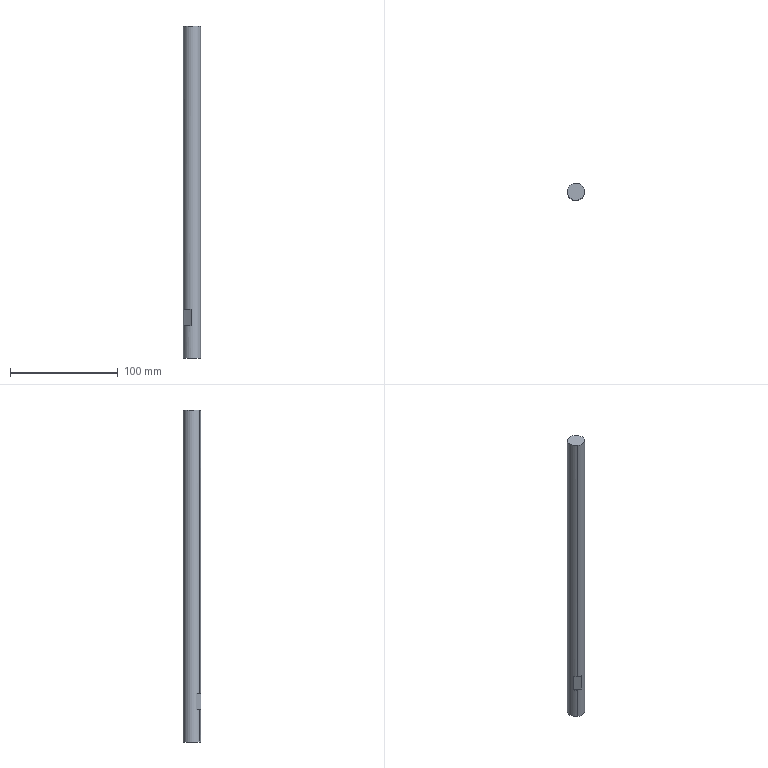Component | SolidWorks | SupportRod-1 | 1 solid | 16 faces | box 16 x 16 x 308 mm | volume 60860 mm3 | plane 8 | cone 4 | cylinder 4 | commonest cylinder face diameters 6.8 x2 16 x2
build123d program:
from build123d import *

# Parameters (mm, degrees)
SKETCH1_W                                            = 8
SKETCH1_H                                            = 308
CUT_EXTRUDE1_DEPTH                                   = 15
CUT_EXTRUDE2_START                                   = -15
CUT_EXTRUDE2_DEPTH                                   = 15
M6_FLAT_HEAD_MACHINE_SCREW_COUNTERSUNK_H_D           = 6.8
M6_FLAT_HEAD_MACHINE_SCREW_COUNTERSUNK_H_DEPTH       = 24.25
M6_FLAT_HEAD_MACHINE_SCREW_COUNTERSUNK_H_CSINK_D     = 8.05
M6_FLAT_HEAD_MACHINE_SCREW_COUNTERSUNK_H_CSINK_ANGLE = 90
M6_FLAT_HEAD_MACHINE_SCREW_COUNTERSUNK_H_TIP         = 2.043


with BuildPart() as part:
    # Sketch1 → Revolve1 (revolve)
    with BuildSketch(Plane.XZ, mode=Mode.PRIVATE) as revolve1_sk:
        with Locations((4, 0)):
            Rectangle(SKETCH1_W, SKETCH1_H)
    revolve(revolve1_sk.sketch.rotate(Axis((0, 0, 154), (0, 0, -1)), 180), axis=Axis((0, 0, 154), (0, 0, -1)))

    # Sketch2 → Cut-Extrude1 (cut)
    with BuildSketch(Plane.XY.offset(124)):
        with BuildLine():
            Line((7, 3.873), (7, -3.873))
            ThreePointArc((7, -3.873), (8, 0), (7, 3.873))
        make_face()
    extrude(amount=-CUT_EXTRUDE1_DEPTH, mode=Mode.SUBTRACT)

    # Sketch3 → Cut-Extrude2 (cut)
    with BuildSketch(Plane(origin=(0, 0, 109), x_dir=(-1, 0, 0), z_dir=(0, 0, -1)).offset(CUT_EXTRUDE2_START)):
        with BuildLine():
            Line((7, 3.873), (7, -3.873))
            ThreePointArc((7, -3.873), (8, 0), (7, 3.873))
        make_face()
    extrude(amount=CUT_EXTRUDE2_DEPTH, mode=Mode.SUBTRACT)

    # M6 Flat Head Machine Screw Countersunk H
    with Locations(Plane.XY.offset(154)):
        with Locations((0, 0)):
            CounterSinkHole(M6_FLAT_HEAD_MACHINE_SCREW_COUNTERSUNK_H_D / 2, M6_FLAT_HEAD_MACHINE_SCREW_COUNTERSUNK_H_CSINK_D / 2, depth=M6_FLAT_HEAD_MACHINE_SCREW_COUNTERSUNK_H_DEPTH, counter_sink_angle=M6_FLAT_HEAD_MACHINE_SCREW_COUNTERSUNK_H_CSINK_ANGLE)
            with Locations((0, 0, -(M6_FLAT_HEAD_MACHINE_SCREW_COUNTERSUNK_H_DEPTH + M6_FLAT_HEAD_MACHINE_SCREW_COUNTERSUNK_H_TIP / 2))):  # 118° drill point
                Cone(0, M6_FLAT_HEAD_MACHINE_SCREW_COUNTERSUNK_H_D / 2, M6_FLAT_HEAD_MACHINE_SCREW_COUNTERSUNK_H_TIP, mode=Mode.SUBTRACT)


solid = part.part

# Placed as in the assembly
solid = solid.moved(Location((-100, -212, -108.5), (180, 0, 125.085)))
STEP:
#1=COLOUR_RGB('',0.7922,0.8196,0.9333);
#2=FILL_AREA_STYLE_COLOUR('',#1);
#3=FILL_AREA_STYLE('',(#2));
#4=SURFACE_STYLE_FILL_AREA(#3);
#5=SURFACE_SIDE_STYLE('',(#4));
#6=SURFACE_STYLE_USAGE(.BOTH.,#5);
#7=PRESENTATION_STYLE_ASSIGNMENT((#6));
#8=CARTESIAN_POINT('',(-3.86,-8.237,-10.31));
#9=VERTEX_POINT('',#8);
#10=CARTESIAN_POINT('',(-4.014,-8.456,-10.31));
#11=VERTEX_POINT('',#10);
#12=CARTESIAN_POINT('',(-3.937,-8.346,-10.31));
#13=DIRECTION('',(0.,0.,-1.));
#14=DIRECTION('',(-0.5748,-0.8183,0.));
#15=AXIS2_PLACEMENT_3D('',#12,#13,#14);
#16=CIRCLE('',#15,0.1339);
#17=EDGE_CURVE('',#9,#11,#16,.T.);
#18=ORIENTED_EDGE('',*,*,#17,.F.);
#19=CARTESIAN_POINT('',(-3.846,-8.217,-10.335));
#20=VERTEX_POINT('',#19);
#21=CARTESIAN_POINT('',(-3.846,-8.217,-10.335));
#22=DIRECTION('',(0.4064,0.5786,-0.7071));
#23=VECTOR('',#22,39.37);
#24=LINE('',#21,#23);
#25=EDGE_CURVE('',#9,#20,#24,.T.);
#26=ORIENTED_EDGE('',*,*,#25,.T.);
#27=CARTESIAN_POINT('',(-4.028,-8.476,-10.335));
#28=VERTEX_POINT('',#27);
#29=CARTESIAN_POINT('',(-3.937,-8.346,-10.335));
#30=DIRECTION('',(0.,0.,-1.));
#31=DIRECTION('',(-0.5748,-0.8183,0.));
#32=AXIS2_PLACEMENT_3D('',#29,#30,#31);
#33=CIRCLE('',#32,0.1585);
#34=EDGE_CURVE('',#20,#28,#33,.T.);
#35=ORIENTED_EDGE('',*,*,#34,.T.);
#36=CARTESIAN_POINT('',(-4.028,-8.476,-10.335));
#37=DIRECTION('',(-0.4064,-0.5786,-0.7071));
#38=VECTOR('',#37,39.37);
#39=LINE('',#36,#38);
#40=EDGE_CURVE('',#11,#28,#39,.T.);
#41=ORIENTED_EDGE('',*,*,#40,.F.);
#42=EDGE_LOOP('',(#18,#26,#35,#41));
#43=FACE_OUTER_BOUND('',#42,.T.);
#44=CARTESIAN_POINT('',(-3.937,-8.346,-10.335));
#45=DIRECTION('',(0.,0.,-1.));
#46=DIRECTION('',(-0.5748,-0.8183,0.));
#47=AXIS2_PLACEMENT_3D('',#44,#45,#46);
#48=CONICAL_SURFACE('',#47,0.1585,0.7854);
#49=ADVANCED_FACE('',(#43),#48,.F.);
#50=CARTESIAN_POINT('',(-3.86,-8.237,-9.38));
#51=VERTEX_POINT('',#50);
#52=CARTESIAN_POINT('',(-4.014,-8.456,-9.38));
#53=VERTEX_POINT('',#52);
#54=CARTESIAN_POINT('',(-3.937,-8.346,-9.38));
#55=DIRECTION('',(0.,0.,-1.));
#56=DIRECTION('',(-0.5748,-0.8183,0.));
#57=AXIS2_PLACEMENT_3D('',#54,#55,#56);
#58=CIRCLE('',#57,0.1339);
#59=EDGE_CURVE('',#51,#53,#58,.T.);
#60=ORIENTED_EDGE('',*,*,#59,.F.);
#61=CARTESIAN_POINT('',(-3.86,-8.237,-10.335));
#62=DIRECTION('',(0.,0.,-1.));
#63=VECTOR('',#62,39.37);
#64=LINE('',#61,#63);
#65=EDGE_CURVE('',#51,#9,#64,.T.);
#66=ORIENTED_EDGE('',*,*,#65,.T.);
#67=ORIENTED_EDGE('',*,*,#17,.T.);
#68=CARTESIAN_POINT('',(-4.014,-8.456,-10.335));
#69=DIRECTION('',(0.,0.,-1.));
#70=VECTOR('',#69,39.37);
#71=LINE('',#68,#70);
#72=EDGE_CURVE('',#53,#11,#71,.T.);
#73=ORIENTED_EDGE('',*,*,#72,.F.);
#74=EDGE_LOOP('',(#60,#66,#67,#73));
#75=FACE_OUTER_BOUND('',#74,.T.);
#76=CARTESIAN_POINT('',(-3.937,-8.346,-10.335));
#77=DIRECTION('',(0.,0.,-1.));
#78=DIRECTION('',(-0.5748,-0.8183,0.));
#79=AXIS2_PLACEMENT_3D('',#76,#77,#78);
#80=CYLINDRICAL_SURFACE('',#79,0.1339);
#81=ADVANCED_FACE('',(#75),#80,.F.);
#82=CARTESIAN_POINT('',(-3.937,-8.346,-9.299));
#83=VERTEX_POINT('',#82);
#84=CARTESIAN_POINT('',(-4.014,-8.456,-9.38));
#85=DIRECTION('',(-0.4927,-0.7014,-0.515));
#86=VECTOR('',#85,39.37);
#87=LINE('',#84,#86);
#88=EDGE_CURVE('',#83,#53,#87,.T.);
#89=ORIENTED_EDGE('',*,*,#88,.F.);
#90=CARTESIAN_POINT('',(-3.86,-8.237,-9.38));
#91=DIRECTION('',(0.4927,0.7014,-0.515));
#92=VECTOR('',#91,39.37);
#93=LINE('',#90,#92);
#94=EDGE_CURVE('',#83,#51,#93,.T.);
#95=ORIENTED_EDGE('',*,*,#94,.T.);
#96=ORIENTED_EDGE('',*,*,#59,.T.);
#97=EDGE_LOOP('',(#89,#95,#96));
#98=FACE_OUTER_BOUND('',#97,.T.);
#99=CARTESIAN_POINT('',(-3.937,-8.346,-9.38));
#100=DIRECTION('',(0.,0.,-1.));
#101=DIRECTION('',(-0.5748,-0.8183,0.));
#102=AXIS2_PLACEMENT_3D('',#99,#100,#101);
#103=CONICAL_SURFACE('',#102,0.1339,1.03);
#104=ADVANCED_FACE('',(#98),#103,.F.);
#105=CARTESIAN_POINT('',(-3.756,-8.089,-10.335));
#106=VERTEX_POINT('',#105);
#107=CARTESIAN_POINT('',(-4.118,-8.604,-10.335));
#108=VERTEX_POINT('',#107);
#109=CARTESIAN_POINT('',(-3.937,-8.346,-10.335));
#110=DIRECTION('',(-0.,0.,1.));
#111=DIRECTION('',(0.5748,0.8183,0.));
#112=AXIS2_PLACEMENT_3D('',#109,#110,#111);
#113=CIRCLE('',#112,0.315);
#114=EDGE_CURVE('',#106,#108,#113,.T.);
#115=ORIENTED_EDGE('',*,*,#114,.T.);
#116=CARTESIAN_POINT('',(-4.118,-8.604,-9.154));
#117=VERTEX_POINT('',#116);
#118=CARTESIAN_POINT('',(-4.118,-8.604,-10.335));
#119=DIRECTION('',(-0.,0.,1.));
#120=VECTOR('',#119,39.37);
#121=LINE('',#118,#120);
#122=EDGE_CURVE('',#108,#117,#121,.T.);
#123=ORIENTED_EDGE('',*,*,#122,.T.);
#124=CARTESIAN_POINT('',(-4.22,-8.484,-9.154));
#125=VERTEX_POINT('',#124);
#126=CARTESIAN_POINT('',(-3.937,-8.346,-9.154));
#127=DIRECTION('',(0.,0.,-1.));
#128=DIRECTION('',(-0.5748,-0.8183,0.));
#129=AXIS2_PLACEMENT_3D('',#126,#127,#128);
#130=CIRCLE('',#129,0.315);
#131=EDGE_CURVE('',#117,#125,#130,.T.);
#132=ORIENTED_EDGE('',*,*,#131,.T.);
#133=CARTESIAN_POINT('',(-4.22,-8.484,-8.563));
#134=VERTEX_POINT('',#133);
#135=CARTESIAN_POINT('',(-4.22,-8.484,-8.563));
#136=DIRECTION('',(0.,0.,-1.));
#137=VECTOR('',#136,39.37);
#138=LINE('',#135,#137);
#139=EDGE_CURVE('',#134,#125,#138,.T.);
#140=ORIENTED_EDGE('',*,*,#139,.F.);
#141=CARTESIAN_POINT('',(-4.118,-8.604,-8.563));
#142=VERTEX_POINT('',#141);
#143=CARTESIAN_POINT('',(-3.937,-8.346,-8.563));
#144=DIRECTION('',(0.,0.,-1.));
#145=DIRECTION('',(-0.5748,-0.8183,0.));
#146=AXIS2_PLACEMENT_3D('',#143,#144,#145);
#147=CIRCLE('',#146,0.315);
#148=EDGE_CURVE('',#142,#134,#147,.T.);
#149=ORIENTED_EDGE('',*,*,#148,.F.);
#150=CARTESIAN_POINT('',(-4.118,-8.604,1.791));
#151=VERTEX_POINT('',#150);
#152=CARTESIAN_POINT('',(-4.118,-8.604,-10.335));
#153=DIRECTION('',(-0.,0.,1.));
#154=VECTOR('',#153,39.37);
#155=LINE('',#152,#154);
#156=EDGE_CURVE('',#142,#151,#155,.T.);
#157=ORIENTED_EDGE('',*,*,#156,.T.);
#158=CARTESIAN_POINT('',(-3.756,-8.089,1.791));
#159=VERTEX_POINT('',#158);
#160=CARTESIAN_POINT('',(-3.937,-8.346,1.791));
#161=DIRECTION('',(-0.,0.,1.));
#162=DIRECTION('',(0.5748,0.8183,0.));
#163=AXIS2_PLACEMENT_3D('',#160,#161,#162);
#164=CIRCLE('',#163,0.315);
#165=EDGE_CURVE('',#159,#151,#164,.T.);
#166=ORIENTED_EDGE('',*,*,#165,.F.);
#167=CARTESIAN_POINT('',(-3.756,-8.089,-8.563));
#168=VERTEX_POINT('',#167);
#169=CARTESIAN_POINT('',(-3.756,-8.089,-10.335));
#170=DIRECTION('',(-0.,0.,1.));
#171=VECTOR('',#170,39.37);
#172=LINE('',#169,#171);
#173=EDGE_CURVE('',#168,#159,#172,.T.);
#174=ORIENTED_EDGE('',*,*,#173,.F.);
#175=CARTESIAN_POINT('',(-3.903,-8.033,-8.563));
#176=VERTEX_POINT('',#175);
#177=CARTESIAN_POINT('',(-3.937,-8.346,-8.563));
#178=DIRECTION('',(-0.,0.,1.));
#179=DIRECTION('',(0.5748,0.8183,0.));
#180=AXIS2_PLACEMENT_3D('',#177,#178,#179);
#181=CIRCLE('',#180,0.315);
#182=EDGE_CURVE('',#168,#176,#181,.T.);
#183=ORIENTED_EDGE('',*,*,#182,.T.);
#184=CARTESIAN_POINT('',(-3.903,-8.033,-9.154));
#185=VERTEX_POINT('',#184);
#186=CARTESIAN_POINT('',(-3.903,-8.033,-9.154));
#187=DIRECTION('',(-0.,0.,1.));
#188=VECTOR('',#187,39.37);
#189=LINE('',#186,#188);
#190=EDGE_CURVE('',#185,#176,#189,.T.);
#191=ORIENTED_EDGE('',*,*,#190,.F.);
#192=CARTESIAN_POINT('',(-3.756,-8.089,-9.154));
#193=VERTEX_POINT('',#192);
#194=CARTESIAN_POINT('',(-3.937,-8.346,-9.154));
#195=DIRECTION('',(-0.,0.,1.));
#196=DIRECTION('',(0.5748,0.8183,0.));
#197=AXIS2_PLACEMENT_3D('',#194,#195,#196);
#198=CIRCLE('',#197,0.315);
#199=EDGE_CURVE('',#193,#185,#198,.T.);
#200=ORIENTED_EDGE('',*,*,#199,.F.);
#201=CARTESIAN_POINT('',(-3.756,-8.089,-10.335));
#202=DIRECTION('',(-0.,0.,1.));
#203=VECTOR('',#202,39.37);
#204=LINE('',#201,#203);
#205=EDGE_CURVE('',#106,#193,#204,.T.);
#206=ORIENTED_EDGE('',*,*,#205,.F.);
#207=EDGE_LOOP('',(#115,#123,#132,#140,#149,#157,#166,#174,#183,#191,#200,#206));
#208=FACE_OUTER_BOUND('',#207,.T.);
#209=CARTESIAN_POINT('',(-3.937,-8.346,-10.335));
#210=DIRECTION('',(-0.,0.,1.));
#211=DIRECTION('',(0.5748,0.8183,0.));
#212=AXIS2_PLACEMENT_3D('',#209,#210,#211);
#213=CYLINDRICAL_SURFACE('',#212,0.315);
#214=ADVANCED_FACE('',(#208),#213,.T.);
#215=ORIENTED_EDGE('',*,*,#122,.F.);
#216=CARTESIAN_POINT('',(-3.937,-8.346,-10.335));
#217=DIRECTION('',(-0.,0.,1.));
#218=DIRECTION('',(0.5748,0.8183,0.));
#219=AXIS2_PLACEMENT_3D('',#216,#217,#218);
#220=CIRCLE('',#219,0.315);
#221=EDGE_CURVE('',#108,#106,#220,.T.);
#222=ORIENTED_EDGE('',*,*,#221,.T.);
#223=ORIENTED_EDGE('',*,*,#205,.T.);
#224=CARTESIAN_POINT('',(-3.654,-8.209,-9.154));
#225=VERTEX_POINT('',#224);
#226=CARTESIAN_POINT('',(-3.937,-8.346,-9.154));
#227=DIRECTION('',(-0.,0.,1.));
#228=DIRECTION('',(0.5748,0.8183,0.));
#229=AXIS2_PLACEMENT_3D('',#226,#227,#228);
#230=CIRCLE('',#229,0.315);
#231=EDGE_CURVE('',#225,#193,#230,.T.);
#232=ORIENTED_EDGE('',*,*,#231,.F.);
#233=CARTESIAN_POINT('',(-3.654,-8.209,-8.563));
#234=VERTEX_POINT('',#233);
#235=CARTESIAN_POINT('',(-3.654,-8.209,-9.154));
#236=DIRECTION('',(-0.,0.,1.));
#237=VECTOR('',#236,39.37);
#238=LINE('',#235,#237);
#239=EDGE_CURVE('',#225,#234,#238,.T.);
#240=ORIENTED_EDGE('',*,*,#239,.T.);
#241=CARTESIAN_POINT('',(-3.937,-8.346,-8.563));
#242=DIRECTION('',(-0.,0.,1.));
#243=DIRECTION('',(0.5748,0.8183,0.));
#244=AXIS2_PLACEMENT_3D('',#241,#242,#243);
#245=CIRCLE('',#244,0.315);
#246=EDGE_CURVE('',#234,#168,#245,.T.);
#247=ORIENTED_EDGE('',*,*,#246,.T.);
#248=ORIENTED_EDGE('',*,*,#173,.T.);
#249=CARTESIAN_POINT('',(-3.937,-8.346,1.791));
#250=DIRECTION('',(-0.,0.,1.));
#251=DIRECTION('',(0.5748,0.8183,0.));
#252=AXIS2_PLACEMENT_3D('',#249,#250,#251);
#253=CIRCLE('',#252,0.315);
#254=EDGE_CURVE('',#151,#159,#253,.T.);
#255=ORIENTED_EDGE('',*,*,#254,.F.);
#256=ORIENTED_EDGE('',*,*,#156,.F.);
#257=CARTESIAN_POINT('',(-3.971,-8.66,-8.563));
#258=VERTEX_POINT('',#257);
#259=CARTESIAN_POINT('',(-3.937,-8.346,-8.563));
#260=DIRECTION('',(0.,0.,-1.));
#261=DIRECTION('',(-0.5748,-0.8183,0.));
#262=AXIS2_PLACEMENT_3D('',#259,#260,#261);
#263=CIRCLE('',#262,0.315);
#264=EDGE_CURVE('',#258,#142,#263,.T.);
#265=ORIENTED_EDGE('',*,*,#264,.F.);
#266=CARTESIAN_POINT('',(-3.971,-8.66,-9.154));
#267=VERTEX_POINT('',#266);
#268=CARTESIAN_POINT('',(-3.971,-8.66,-8.563));
#269=DIRECTION('',(0.,0.,-1.));
#270=VECTOR('',#269,39.37);
#271=LINE('',#268,#270);
#272=EDGE_CURVE('',#258,#267,#271,.T.);
#273=ORIENTED_EDGE('',*,*,#272,.T.);
#274=CARTESIAN_POINT('',(-3.937,-8.346,-9.154));
#275=DIRECTION('',(0.,0.,-1.));
#276=DIRECTION('',(-0.5748,-0.8183,0.));
#277=AXIS2_PLACEMENT_3D('',#274,#275,#276);
#278=CIRCLE('',#277,0.315);
#279=EDGE_CURVE('',#267,#117,#278,.T.);
#280=ORIENTED_EDGE('',*,*,#279,.T.);
#281=EDGE_LOOP('',(#215,#222,#223,#232,#240,#247,#248,#255,#256,#265,#273,#280));
#282=FACE_OUTER_BOUND('',#281,.T.);
#283=CARTESIAN_POINT('',(-3.937,-8.346,-10.335));
#284=DIRECTION('',(-0.,0.,1.));
#285=DIRECTION('',(0.5748,0.8183,0.));
#286=AXIS2_PLACEMENT_3D('',#283,#284,#285);
#287=CYLINDRICAL_SURFACE('',#286,0.315);
#288=ADVANCED_FACE('',(#282),#287,.T.);
#289=CARTESIAN_POINT('',(-3.937,-8.346,-10.335));
#290=DIRECTION('',(0.,0.,-1.));
#291=DIRECTION('',(-0.5748,-0.8183,0.));
#292=AXIS2_PLACEMENT_3D('',#289,#290,#291);
#293=CIRCLE('',#292,0.1585);
#294=EDGE_CURVE('',#28,#20,#293,.T.);
#295=ORIENTED_EDGE('',*,*,#294,.F.);
#296=ORIENTED_EDGE('',*,*,#34,.F.);
#297=EDGE_LOOP('',(#295,#296));
#298=FACE_BOUND('',#297,.T.);
#299=ORIENTED_EDGE('',*,*,#114,.F.);
#300=ORIENTED_EDGE('',*,*,#221,.F.);
#301=EDGE_LOOP('',(#299,#300));
#302=FACE_OUTER_BOUND('',#301,.T.);
#303=CARTESIAN_POINT('',(-4.118,-8.604,-10.335));
#304=DIRECTION('',(0.,0.,-1.));
#305=DIRECTION('',(-0.5748,-0.8183,-0.));
#306=AXIS2_PLACEMENT_3D('',#303,#304,#305);
#307=PLANE('',#306);
#308=ADVANCED_FACE('',(#298,#302),#307,.T.);
#309=ORIENTED_EDGE('',*,*,#165,.T.);
#310=ORIENTED_EDGE('',*,*,#254,.T.);
#311=EDGE_LOOP('',(#309,#310));
#312=FACE_OUTER_BOUND('',#311,.T.);
#313=CARTESIAN_POINT('',(-3.937,-8.346,1.791));
#314=DIRECTION('',(-0.,-0.,1.));
#315=DIRECTION('',(0.5748,0.8183,0.));
#316=AXIS2_PLACEMENT_3D('',#313,#314,#315);
#317=PLANE('',#316);
#318=ADVANCED_FACE('',(#312),#317,.T.);
#319=CARTESIAN_POINT('',(-4.22,-8.484,-9.154));
#320=DIRECTION('',(0.8183,-0.5748,0.));
#321=VECTOR('',#320,39.37);
#322=LINE('',#319,#321);
#323=EDGE_CURVE('',#125,#267,#322,.T.);
#324=ORIENTED_EDGE('',*,*,#323,.T.);
#325=ORIENTED_EDGE('',*,*,#272,.F.);
#326=CARTESIAN_POINT('',(-4.22,-8.484,-8.563));
#327=DIRECTION('',(0.8183,-0.5748,0.));
#328=VECTOR('',#327,39.37);
#329=LINE('',#326,#328);
#330=EDGE_CURVE('',#134,#258,#329,.T.);
#331=ORIENTED_EDGE('',*,*,#330,.F.);
#332=ORIENTED_EDGE('',*,*,#139,.T.);
#333=EDGE_LOOP('',(#324,#325,#331,#332));
#334=FACE_OUTER_BOUND('',#333,.T.);
#335=CARTESIAN_POINT('',(-4.22,-8.484,-8.563));
#336=DIRECTION('',(0.5748,0.8183,0.));
#337=DIRECTION('',(0.,0.,-1.));
#338=AXIS2_PLACEMENT_3D('',#335,#336,#337);
#339=PLANE('',#338);
#340=ADVANCED_FACE('',(#334),#339,.F.);
#341=ORIENTED_EDGE('',*,*,#264,.T.);
#342=ORIENTED_EDGE('',*,*,#148,.T.);
#343=ORIENTED_EDGE('',*,*,#330,.T.);
#344=EDGE_LOOP('',(#341,#342,#343));
#345=FACE_OUTER_BOUND('',#344,.T.);
#346=CARTESIAN_POINT('',(-3.937,-8.346,-8.563));
#347=DIRECTION('',(0.,0.,-1.));
#348=DIRECTION('',(-0.5748,-0.8183,-0.));
#349=AXIS2_PLACEMENT_3D('',#346,#347,#348);
#350=PLANE('',#349);
#351=ADVANCED_FACE('',(#345),#350,.T.);
#352=ORIENTED_EDGE('',*,*,#279,.F.);
#353=ORIENTED_EDGE('',*,*,#323,.F.);
#354=ORIENTED_EDGE('',*,*,#131,.F.);
#355=EDGE_LOOP('',(#352,#353,#354));
#356=FACE_OUTER_BOUND('',#355,.T.);
#357=CARTESIAN_POINT('',(-3.937,-8.346,-9.154));
#358=DIRECTION('',(0.,0.,-1.));
#359=DIRECTION('',(-0.5748,-0.8183,-0.));
#360=AXIS2_PLACEMENT_3D('',#357,#358,#359);
#361=PLANE('',#360);
#362=ADVANCED_FACE('',(#356),#361,.F.);
#363=CARTESIAN_POINT('',(-3.903,-8.033,-8.563));
#364=DIRECTION('',(0.8183,-0.5748,0.));
#365=VECTOR('',#364,39.37);
#366=LINE('',#363,#365);
#367=EDGE_CURVE('',#176,#234,#366,.T.);
#368=ORIENTED_EDGE('',*,*,#367,.T.);
#369=ORIENTED_EDGE('',*,*,#239,.F.);
#370=CARTESIAN_POINT('',(-3.903,-8.033,-9.154));
#371=DIRECTION('',(0.8183,-0.5748,0.));
#372=VECTOR('',#371,39.37);
#373=LINE('',#370,#372);
#374=EDGE_CURVE('',#185,#225,#373,.T.);
#375=ORIENTED_EDGE('',*,*,#374,.F.);
#376=ORIENTED_EDGE('',*,*,#190,.T.);
#377=EDGE_LOOP('',(#368,#369,#375,#376));
#378=FACE_OUTER_BOUND('',#377,.T.);
#379=CARTESIAN_POINT('',(-3.903,-8.033,-9.154));
#380=DIRECTION('',(-0.5748,-0.8183,-0.));
#381=DIRECTION('',(-0.8183,0.5748,-0.));
#382=AXIS2_PLACEMENT_3D('',#379,#380,#381);
#383=PLANE('',#382);
#384=ADVANCED_FACE('',(#378),#383,.F.);
#385=ORIENTED_EDGE('',*,*,#231,.T.);
#386=ORIENTED_EDGE('',*,*,#199,.T.);
#387=ORIENTED_EDGE('',*,*,#374,.T.);
#388=EDGE_LOOP('',(#385,#386,#387));
#389=FACE_OUTER_BOUND('',#388,.T.);
#390=CARTESIAN_POINT('',(-3.937,-8.346,-9.154));
#391=DIRECTION('',(-0.,-0.,1.));
#392=DIRECTION('',(0.5748,0.8183,0.));
#393=AXIS2_PLACEMENT_3D('',#390,#391,#392);
#394=PLANE('',#393);
#395=ADVANCED_FACE('',(#389),#394,.T.);
#396=ORIENTED_EDGE('',*,*,#246,.F.);
#397=ORIENTED_EDGE('',*,*,#367,.F.);
#398=ORIENTED_EDGE('',*,*,#182,.F.);
#399=EDGE_LOOP('',(#396,#397,#398));
#400=FACE_OUTER_BOUND('',#399,.T.);
#401=CARTESIAN_POINT('',(-3.937,-8.346,-8.563));
#402=DIRECTION('',(-0.,-0.,1.));
#403=DIRECTION('',(0.5748,0.8183,0.));
#404=AXIS2_PLACEMENT_3D('',#401,#402,#403);
#405=PLANE('',#404);
#406=ADVANCED_FACE('',(#400),#405,.F.);
#407=ORIENTED_EDGE('',*,*,#94,.F.);
#408=ORIENTED_EDGE('',*,*,#88,.T.);
#409=CARTESIAN_POINT('',(-3.937,-8.346,-9.38));
#410=DIRECTION('',(0.,0.,-1.));
#411=DIRECTION('',(-0.5748,-0.8183,0.));
#412=AXIS2_PLACEMENT_3D('',#409,#410,#411);
#413=CIRCLE('',#412,0.1339);
#414=EDGE_CURVE('',#53,#51,#413,.T.);
#415=ORIENTED_EDGE('',*,*,#414,.T.);
#416=EDGE_LOOP('',(#407,#408,#415));
#417=FACE_OUTER_BOUND('',#416,.T.);
#418=CARTESIAN_POINT('',(-3.937,-8.346,-9.38));
#419=DIRECTION('',(0.,0.,-1.));
#420=DIRECTION('',(-0.5748,-0.8183,0.));
#421=AXIS2_PLACEMENT_3D('',#418,#419,#420);
#422=CONICAL_SURFACE('',#421,0.1339,1.03);
#423=ADVANCED_FACE('',(#417),#422,.F.);
#424=ORIENTED_EDGE('',*,*,#65,.F.);
#425=ORIENTED_EDGE('',*,*,#414,.F.);
#426=ORIENTED_EDGE('',*,*,#72,.T.);
#427=CARTESIAN_POINT('',(-3.937,-8.346,-10.31));
#428=DIRECTION('',(0.,0.,-1.));
#429=DIRECTION('',(-0.5748,-0.8183,0.));
#430=AXIS2_PLACEMENT_3D('',#427,#428,#429);
#431=CIRCLE('',#430,0.1339);
#432=EDGE_CURVE('',#11,#9,#431,.T.);
#433=ORIENTED_EDGE('',*,*,#432,.T.);
#434=EDGE_LOOP('',(#424,#425,#426,#433));
#435=FACE_OUTER_BOUND('',#434,.T.);
#436=CARTESIAN_POINT('',(-3.937,-8.346,-10.335));
#437=DIRECTION('',(0.,0.,-1.));
#438=DIRECTION('',(-0.5748,-0.8183,0.));
#439=AXIS2_PLACEMENT_3D('',#436,#437,#438);
#440=CYLINDRICAL_SURFACE('',#439,0.1339);
#441=ADVANCED_FACE('',(#435),#440,.F.);
#442=ORIENTED_EDGE('',*,*,#25,.F.);
#443=ORIENTED_EDGE('',*,*,#432,.F.);
#444=ORIENTED_EDGE('',*,*,#40,.T.);
#445=ORIENTED_EDGE('',*,*,#294,.T.);
#446=EDGE_LOOP('',(#442,#443,#444,#445));
#447=FACE_OUTER_BOUND('',#446,.T.);
#448=CARTESIAN_POINT('',(-3.937,-8.346,-10.335));
#449=DIRECTION('',(0.,0.,-1.));
#450=DIRECTION('',(-0.5748,-0.8183,0.));
#451=AXIS2_PLACEMENT_3D('',#448,#449,#450);
#452=CONICAL_SURFACE('',#451,0.1585,0.7854);
#453=ADVANCED_FACE('',(#447),#452,.F.);
#454=CLOSED_SHELL('',(#49,#81,#104,#214,#288,#308,#318,#340,#351,#362,#384,#395,#406,#423,#441,#453));
#455=MANIFOLD_SOLID_BREP('',#454);
#456=STYLED_ITEM('',(#7),#455);
#457=PRESENTATION_LAYER_ASSIGNMENT('','',(#456));
#458=(LENGTH_UNIT()NAMED_UNIT(*)SI_UNIT($,.METRE.));
#459=LENGTH_MEASURE_WITH_UNIT(LENGTH_MEASURE(0.0254),#458);
#460=DIMENSIONAL_EXPONENTS(1.,0.,0.,0.,0.,0.,0.);
#461=(CONVERSION_BASED_UNIT('',#459)LENGTH_UNIT()NAMED_UNIT(#460));
#462=UNCERTAINTY_MEASURE_WITH_UNIT(LENGTH_MEASURE(0.00001),#461,'','');
#463=(NAMED_UNIT(*)PLANE_ANGLE_UNIT()SI_UNIT($,.RADIAN.));
#464=(NAMED_UNIT(*)SI_UNIT($,.STERADIAN.)SOLID_ANGLE_UNIT());
#465=(GEOMETRIC_REPRESENTATION_CONTEXT(3)GLOBAL_UNCERTAINTY_ASSIGNED_CONTEXT((#462))GLOBAL_UNIT_ASSIGNED_CONTEXT((#461,#463,#464))REPRESENTATION_CONTEXT('',''));
#466=MECHANICAL_DESIGN_GEOMETRIC_PRESENTATION_REPRESENTATION('',(#456),#465);
#467=CARTESIAN_POINT('',(0.,0.,0.));
#468=DIRECTION('',(0.,0.,1.));
#469=DIRECTION('',(1.,0.,0.));
#470=AXIS2_PLACEMENT_3D('',#467,#468,#469);
#471=(LENGTH_UNIT()NAMED_UNIT(*)SI_UNIT($,.METRE.));
#472=LENGTH_MEASURE_WITH_UNIT(LENGTH_MEASURE(0.0254),#471);
#473=DIMENSIONAL_EXPONENTS(1.,0.,0.,0.,0.,0.,0.);
#474=(CONVERSION_BASED_UNIT('',#472)LENGTH_UNIT()NAMED_UNIT(#473));
#475=UNCERTAINTY_MEASURE_WITH_UNIT(LENGTH_MEASURE(0.00001),#474,'','');
#476=(NAMED_UNIT(*)PLANE_ANGLE_UNIT()SI_UNIT($,.RADIAN.));
#477=(NAMED_UNIT(*)SI_UNIT($,.STERADIAN.)SOLID_ANGLE_UNIT());
#478=(GEOMETRIC_REPRESENTATION_CONTEXT(3)GLOBAL_UNCERTAINTY_ASSIGNED_CONTEXT((#475))GLOBAL_UNIT_ASSIGNED_CONTEXT((#474,#476,#477))REPRESENTATION_CONTEXT('',''));
#479=ADVANCED_BREP_SHAPE_REPRESENTATION('',(#455,#470),#478);